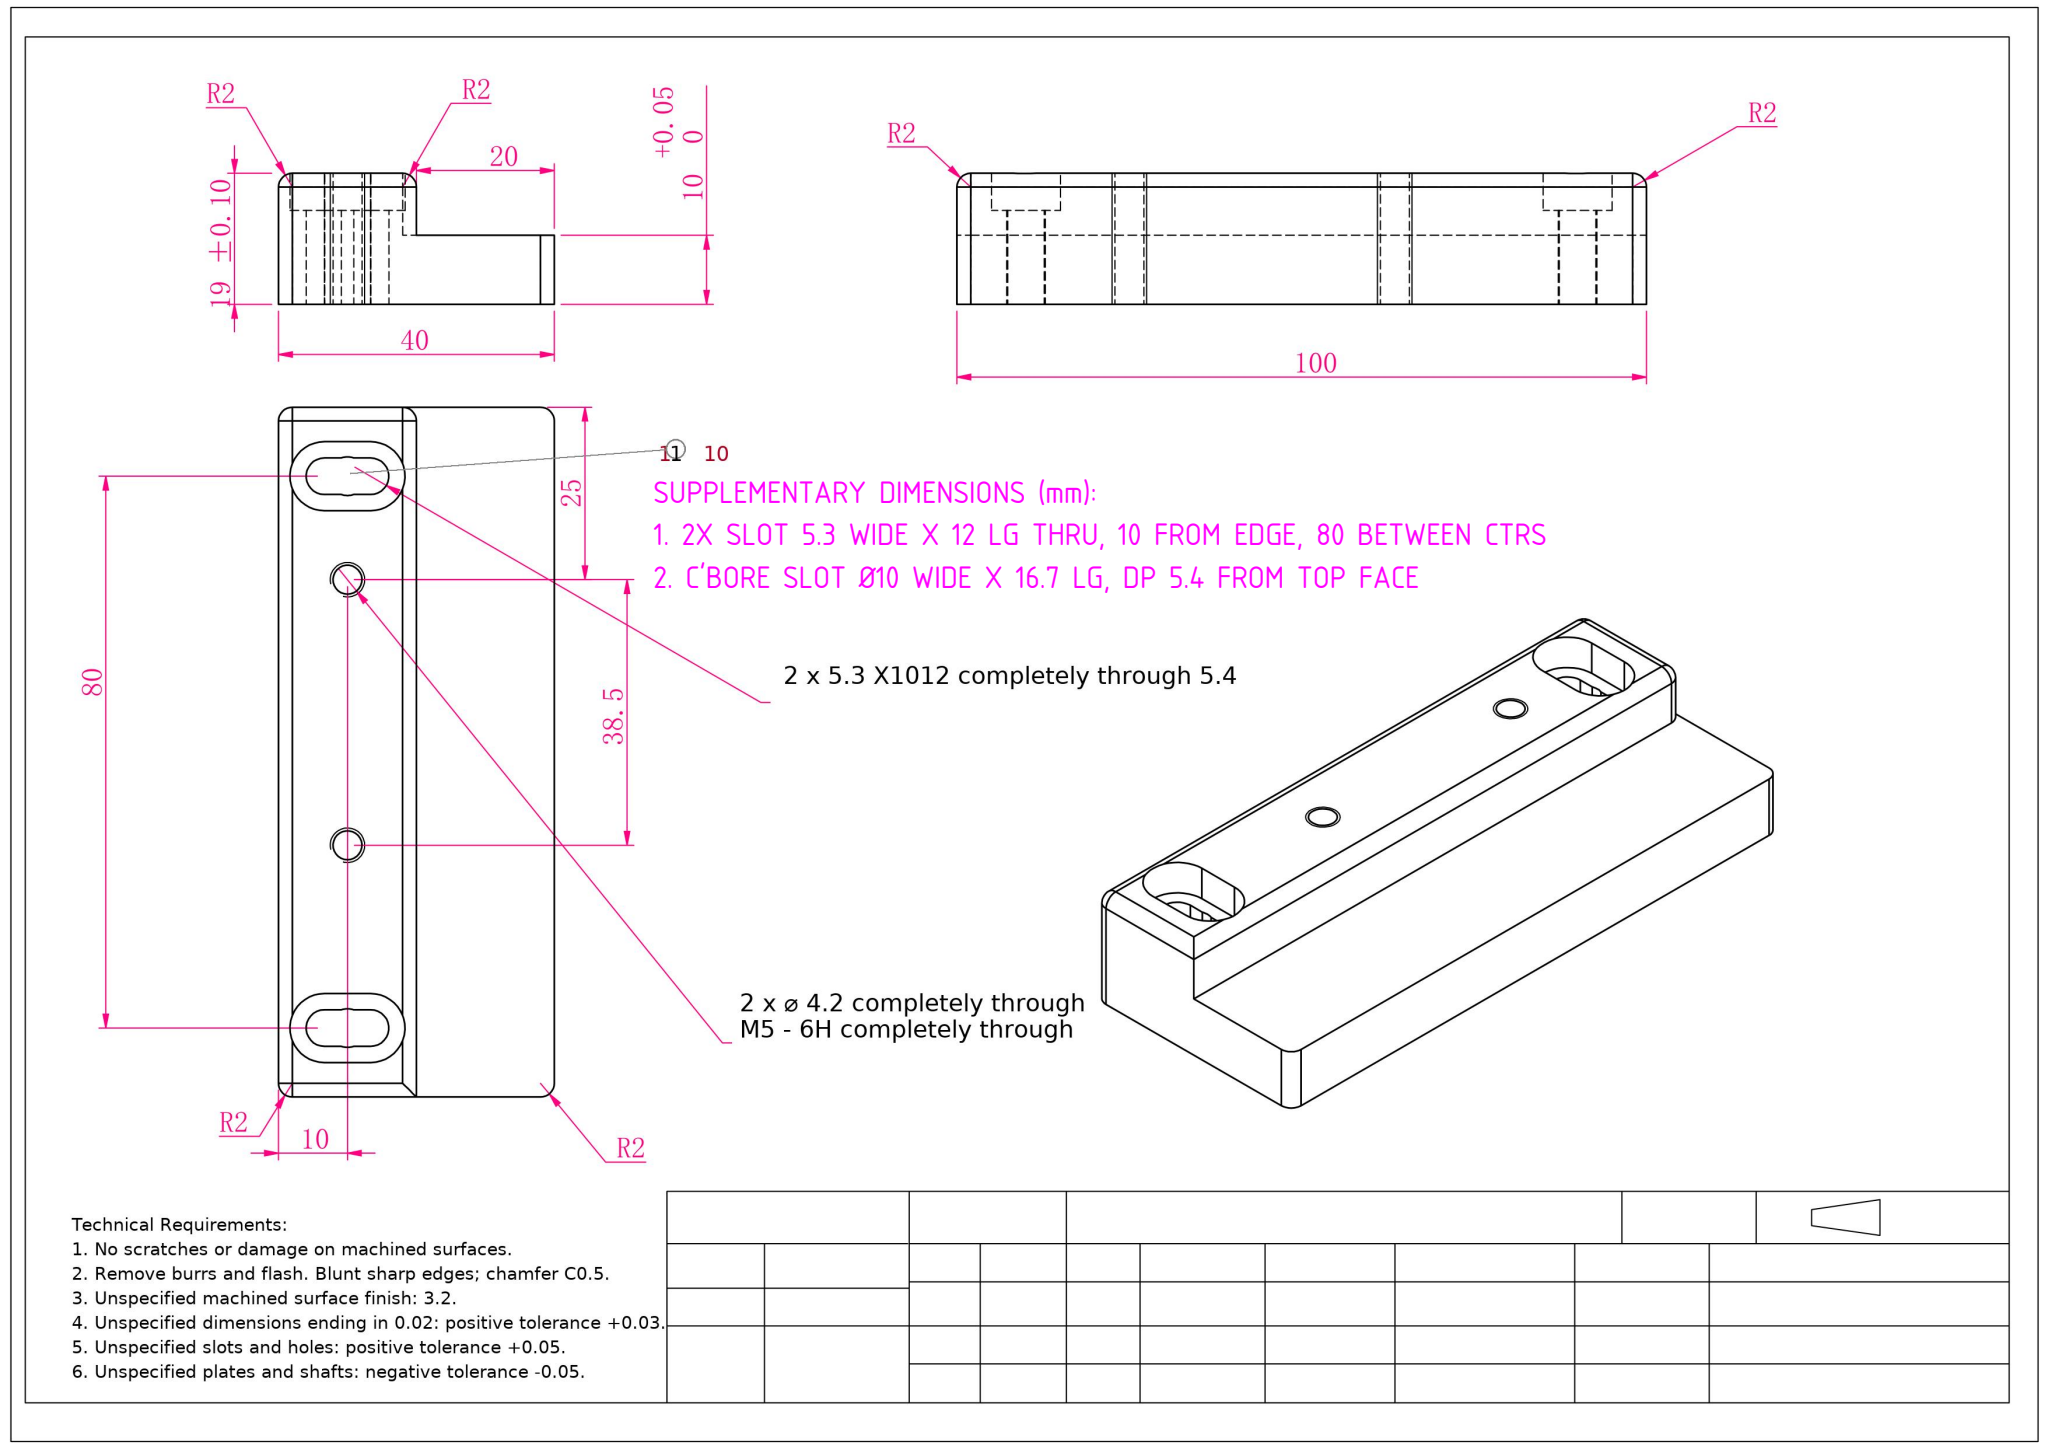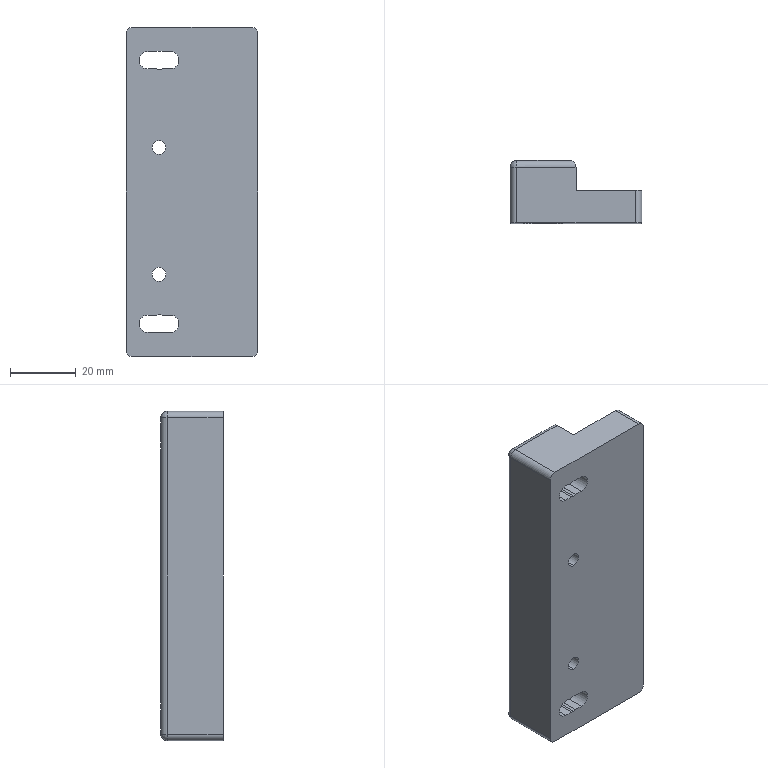Part | SolidWorks | mm | 1 solid | 54 faces | box 40 x 19 x 100 mm | volume 54067 mm3 | cylinder 27 | plane 24 | sphere 3 | commonest cylinder face diameters 4 x9 5.6 x6 4.2 x4 5.3 x4 10 x4